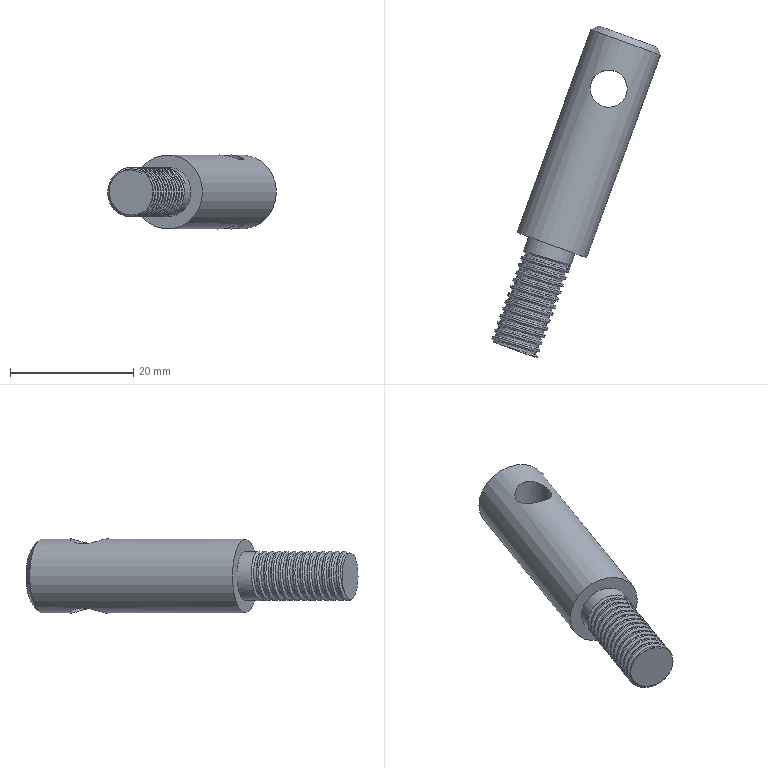Component | NX | 6 | 1 solid | 23 faces | volume 4489 mm3 | cylinder 16 | plane 4 | spline 2 | cone 1 | commonest cylinder face diameters 8 x13 12 x1 7.18 x1 6 x1